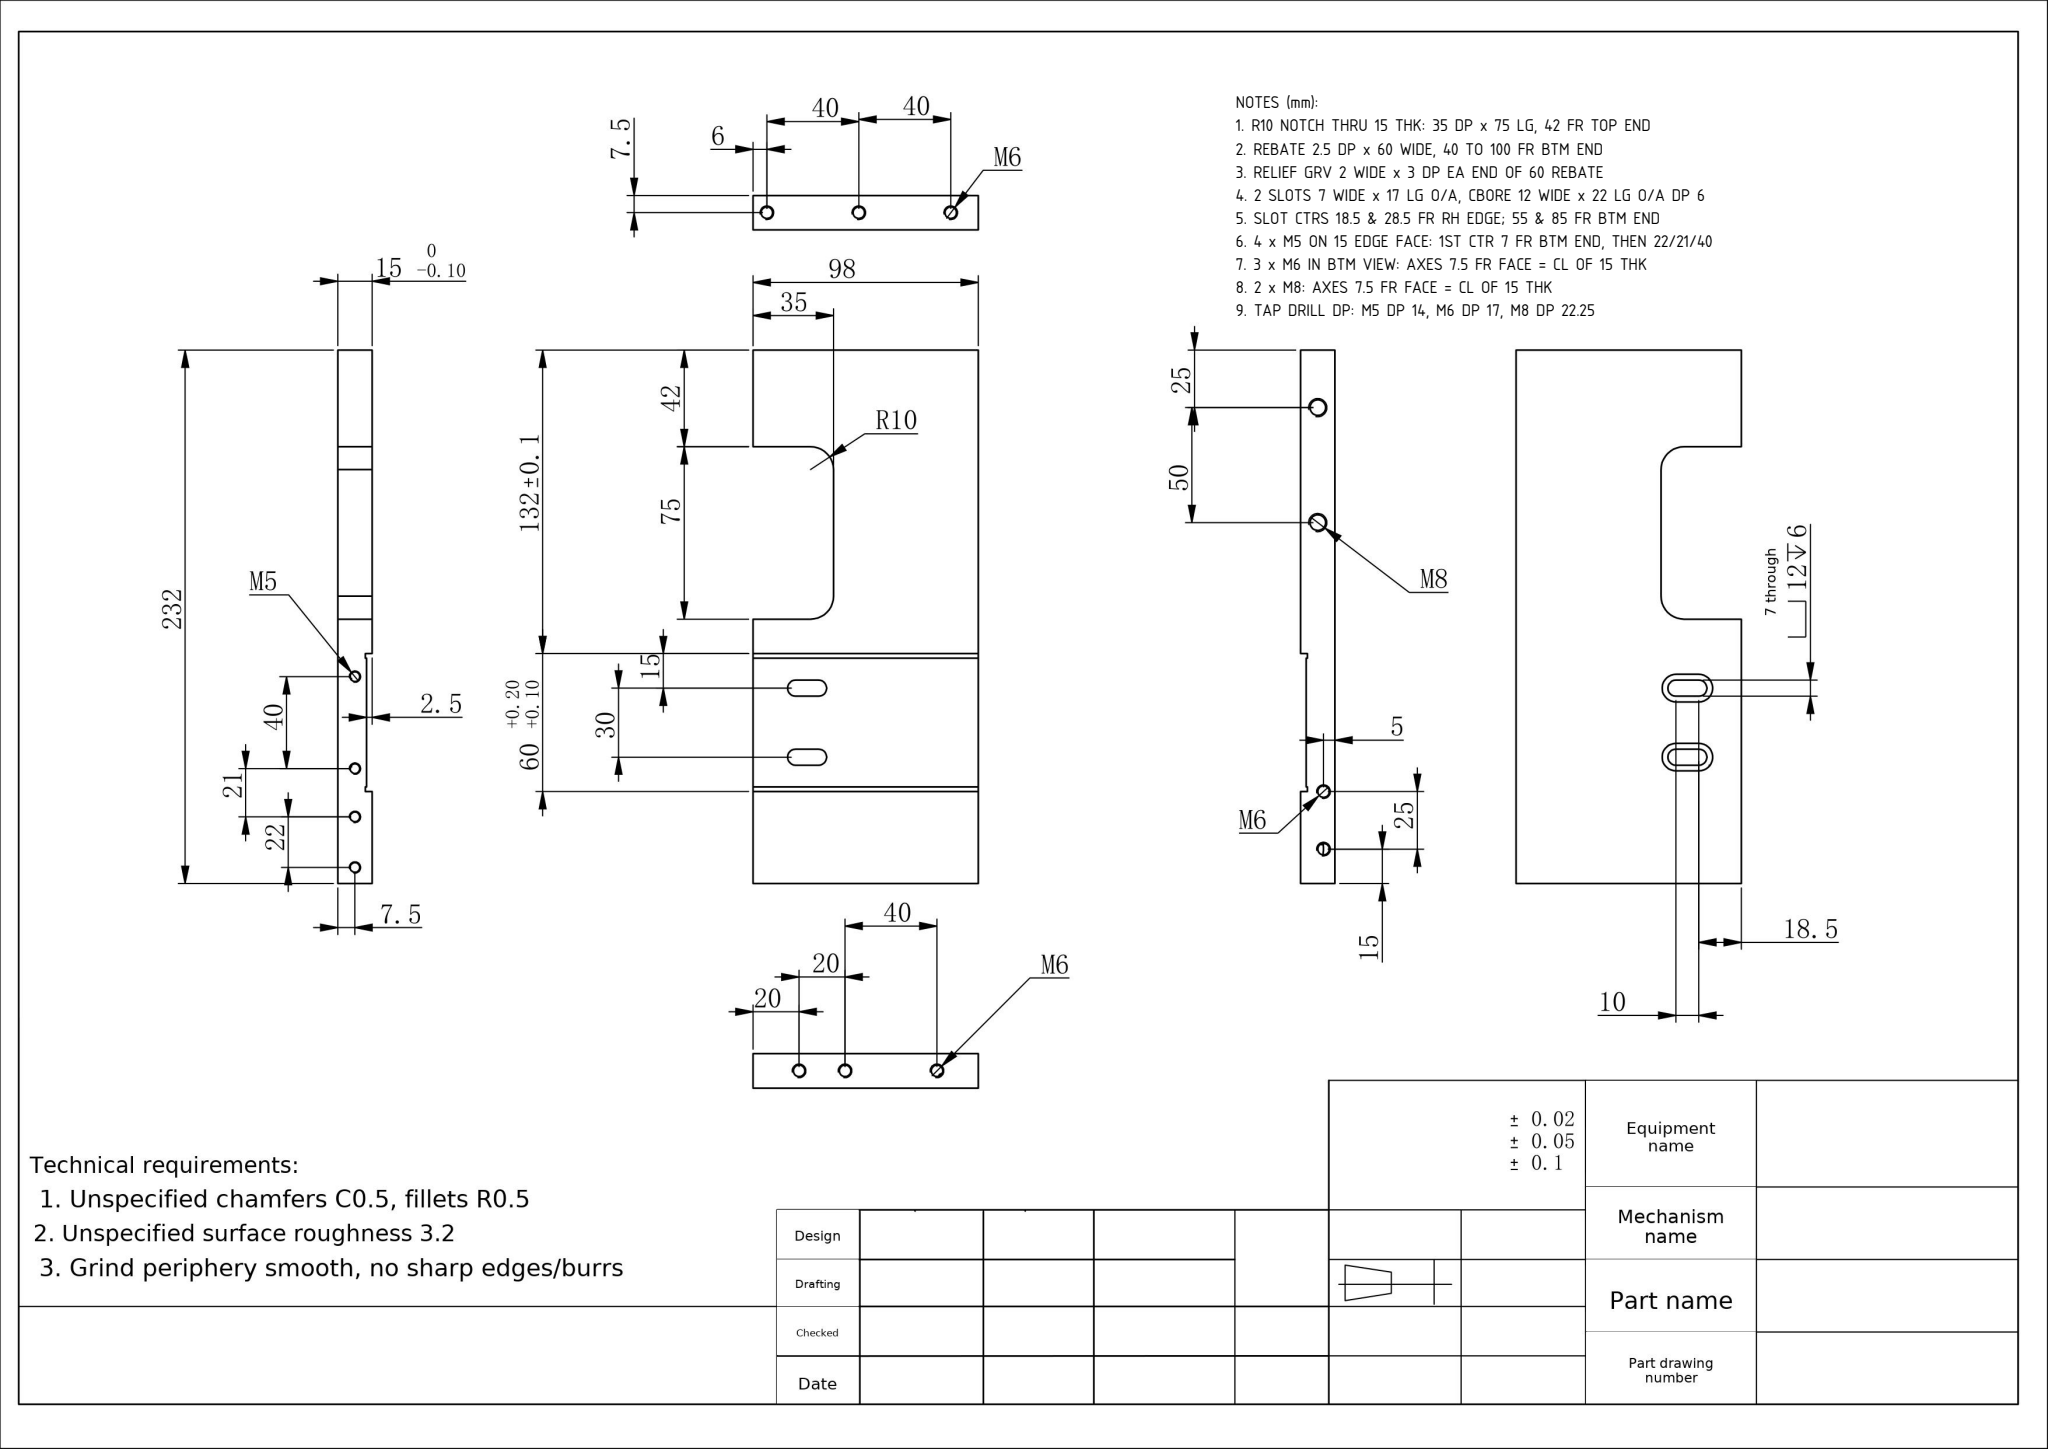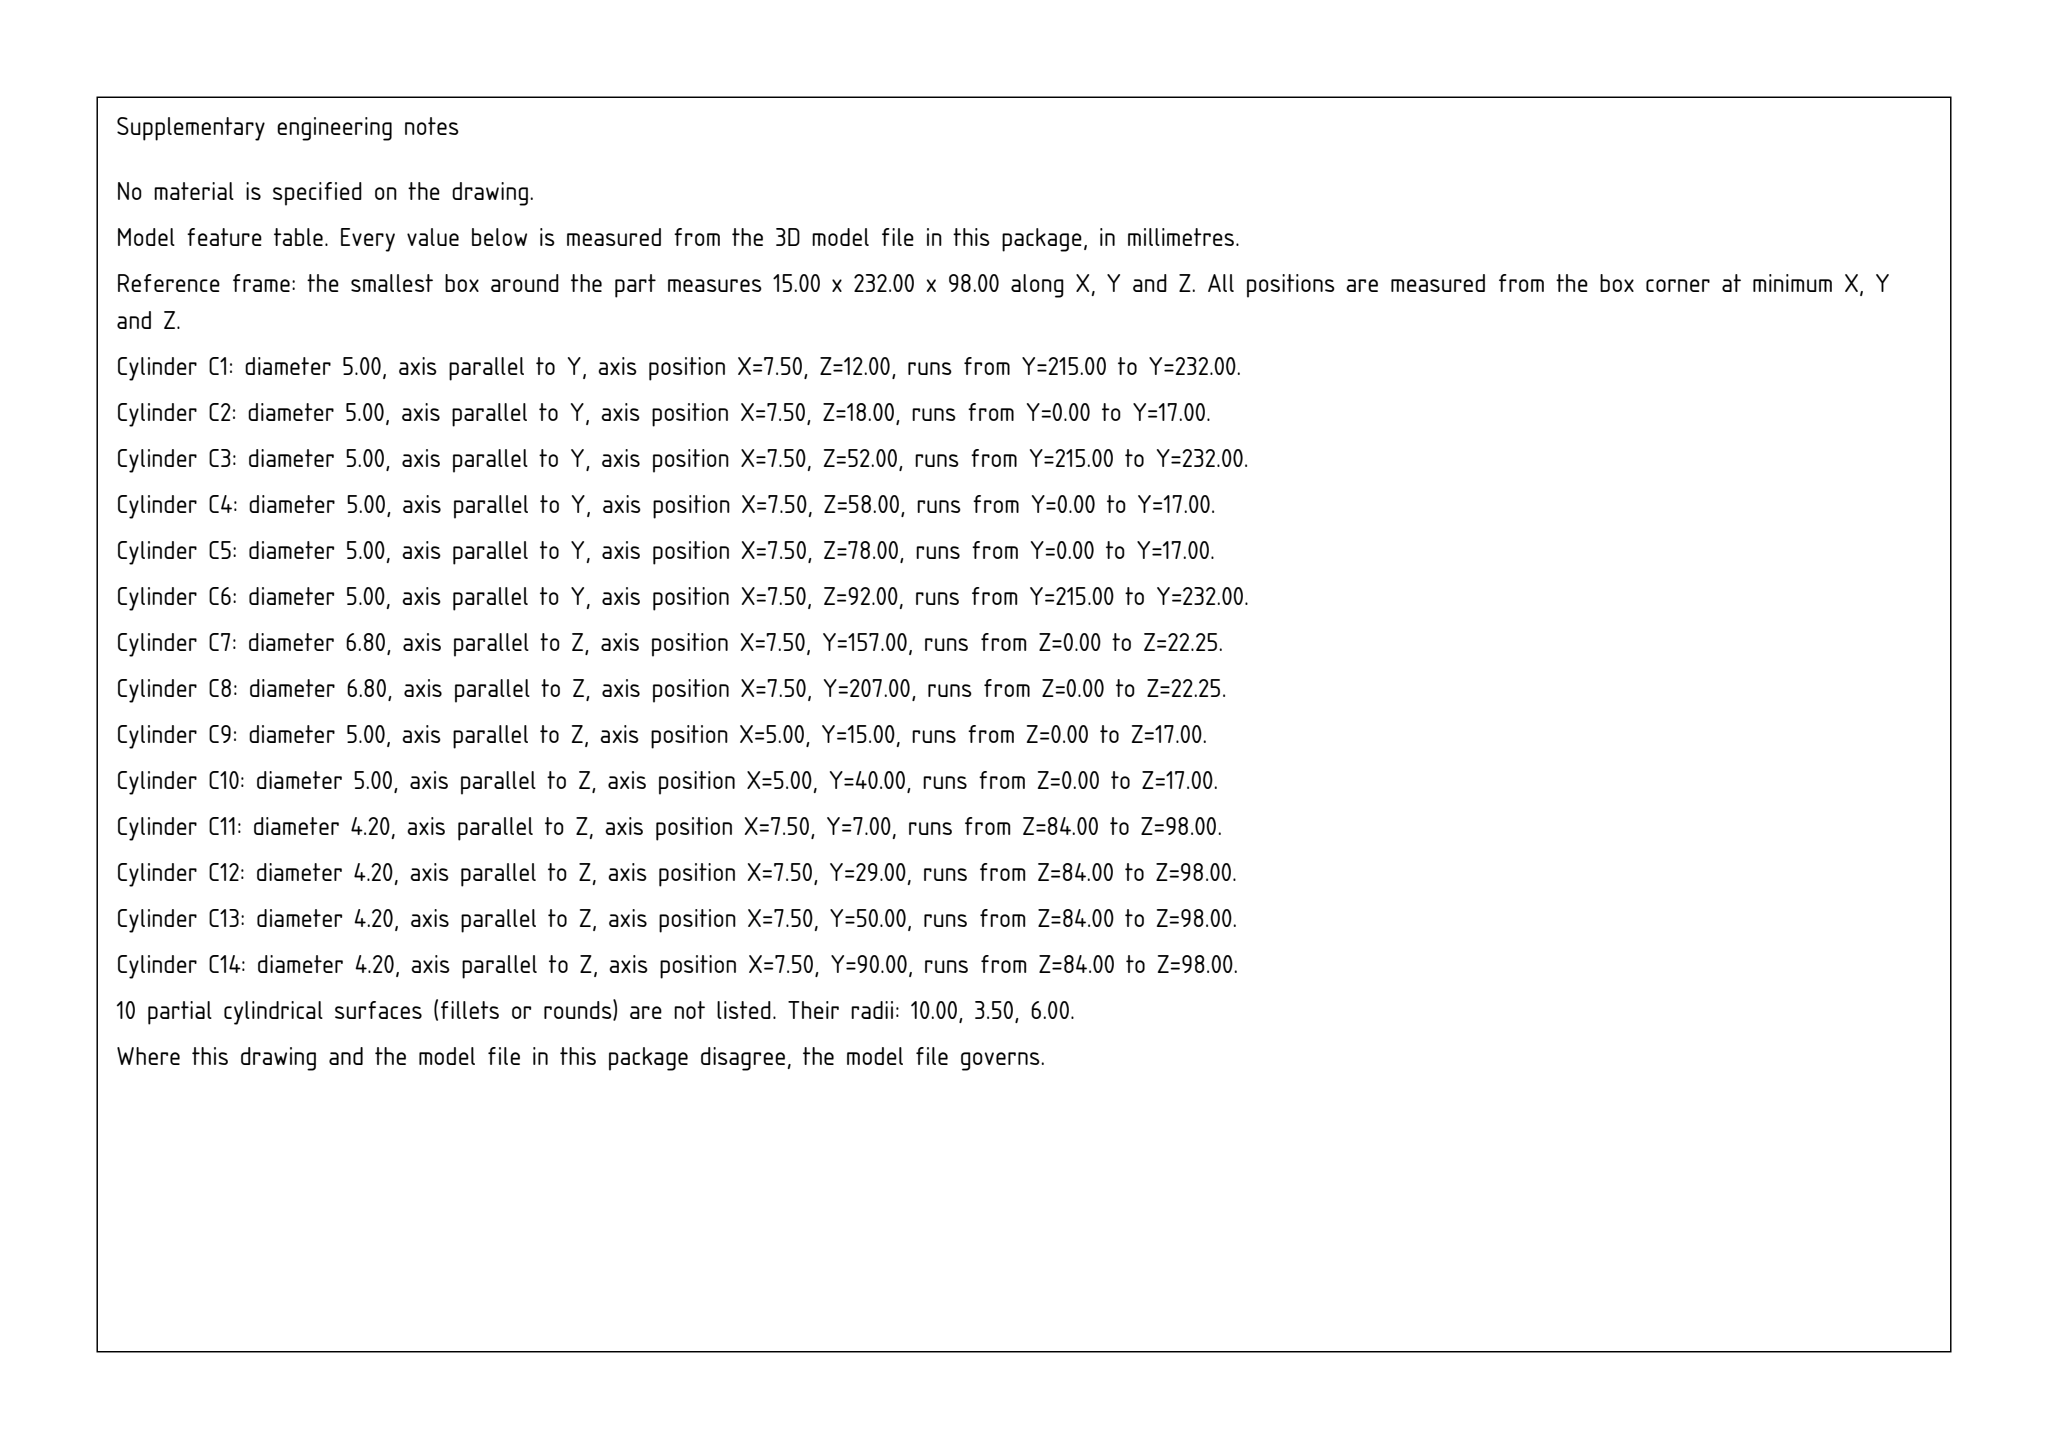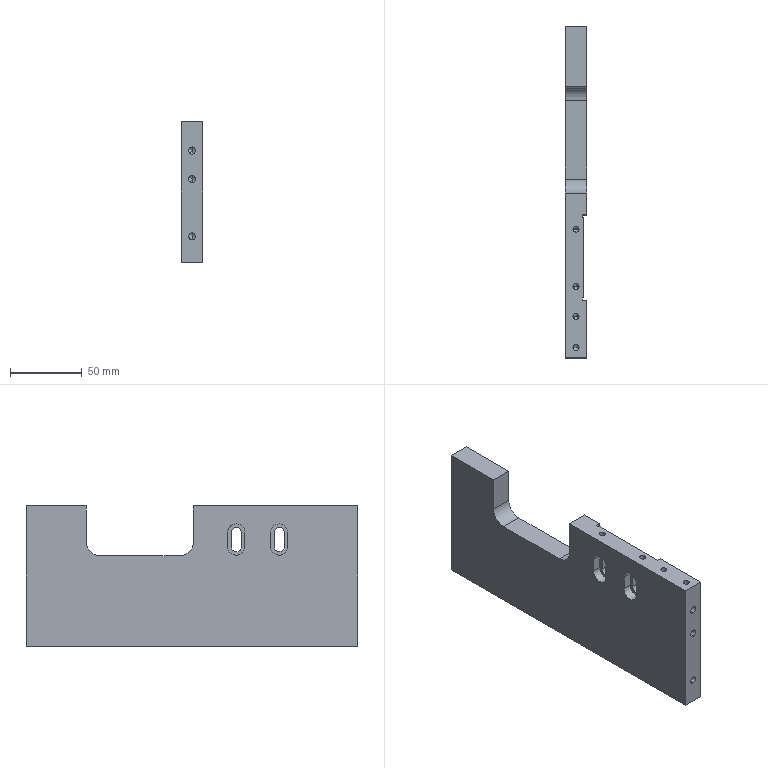Part | SolidWorks | mm | 1 solid | 99 faces | box 15 x 232 x 98 mm | volume 278005 mm3 | cylinder 43 | cone 28 | plane 28 | commonest cylinder face diameters 5 x17 4.2 x8 12 x6 7 x6 6.8 x4 20 x2
Drawing notes:
R10 NOTCH THRU 15 THK: 35 DP x 75 LG, 42 FR TOP END | from the solid: R10 cyls len 15 = full thk; z 63-98 = 35; y 115-190 = 75; 232-190 = 42
REBATE 2.5 DP x 60 WIDE, 40 TO 100 FR BTM END | from the solid: x planes 15 & 12.5 -> 2.5 dp; y planes 40 & 100 -> 60 wide, 40 fr y=0
RELIEF GRV 2 WIDE x 3 DP EA END OF 60 REBATE | from the solid: x plane 12 (2 faces) = 3 dp; y planes 40/42 and 98/100 -> 2 wide
2 SLOTS 7 WIDE x 17 LG O/A, CBORE 12 WIDE x 22 LG O/A DP 6 | from the solid: Ø7 x-axis cyls z=69.5 & 79.5 (10 apart) -> 17 o/a; Ø12 cbore len 6 -> 22 o/a
SLOT CTRS 18.5 & 28.5 FR RH EDGE; 55 & 85 FR BTM END | from the solid: hole axes z=79.5 & 69.5 of 98; y=55 & 85 of 232
4 x M5 ON 15 EDGE FACE: 1ST CTR 7 FR BTM END, THEN 22/21/40 | from the solid: Ø4.2 z-axis holes at y=7,29,50,90, x=7.5 (M5 tap drills)
3 x M6 IN BTM VIEW: AXES 7.5 FR FACE = CL OF 15 THK | from the solid: Ø5.0 y-axis cyls at x=7.5; bbox x=15.0 so 7.5 = mid-thk
2 x M8: AXES 7.5 FR FACE = CL OF 15 THK | from the solid: Ø6.8 z-axis holes at x=7.5, y=157 & 207; bbox x=15
TAP DRILL DP: M5 DP 14, M6 DP 17, M8 DP 22.25 | from the solid: Ø4.2 L=14, Ø5.0 L=17, Ø6.8 L=22.25 cylinders
build123d program:
from build123d import *

# Parameters (mm, degrees)
SKETCH1_W             = 98
SKETCH1_H             = 232
BOSS_EXTRUDE1_DEPTH   = 15
CUT_EXTRUDE1_DEPTH    = 253.295
SKETCH3_W             = 2.5
SKETCH3_H             = 60
CUT_EXTRUDE2_DEPTH    = 120
SKETCH4_W             = 98
SKETCH4_H             = 2
CUT_EXTRUDE3_DEPTH    = 0.5
M6_TAPPED_HOLE1_D     = 5
M6_TAPPED_HOLE1_DEPTH = 17
M6_TAPPED_HOLE1_TIP   = 1.502
M5_TAPPED_HOLE1_D     = 4.2
M5_TAPPED_HOLE1_DEPTH = 14
M5_TAPPED_HOLE1_TIP   = 1.262
M5_TAPPED_HOLE2_D     = 4.2
M5_TAPPED_HOLE2_DEPTH = 14
M5_TAPPED_HOLE2_TIP   = 1.262
M6_TAPPED_HOLE2_D     = 5
M6_TAPPED_HOLE2_DEPTH = 17
M6_TAPPED_HOLE2_TIP   = 1.502
M6_TAPPED_HOLE3_D     = 5
M6_TAPPED_HOLE3_DEPTH = 17
M6_TAPPED_HOLE3_TIP   = 1.502
CUT_EXTRUDE4_DEPTH    = 30
CUT_EXTRUDE5_DEPTH    = 6
M8_TAPPED_HOLE2_D     = 6.8
M8_TAPPED_HOLE2_DEPTH = 22.25
M8_TAPPED_HOLE2_TIP   = 2.043


with BuildPart() as part:
    # Sketch1 → Boss-Extrude1 (new body)
    with BuildSketch(Plane(origin=(0, 0, 0), x_dir=(0, 0, -1), z_dir=(1, 0, 0))):
        with Locations((49, 116)):
            Rectangle(SKETCH1_W, SKETCH1_H)
    extrude(amount=BOSS_EXTRUDE1_DEPTH)

    # Sketch2 → Cut-Extrude1 (cut, through all)
    with BuildSketch(Plane.ZY):
        with BuildLine():
            Line((0, 115), (-25, 115))
            ThreePointArc((-25, 115), (-32.071, 117.929), (-35, 125))
            Line((-35, 125), (-35, 180))
            ThreePointArc((-35, 180), (-32.071, 187.071), (-25, 190))
            Line((-25, 190), (0, 190))
            Line((0, 190), (0, 115))
        make_face()
    extrude(amount=-CUT_EXTRUDE1_DEPTH, mode=Mode.SUBTRACT)

    # Sketch3 → Cut-Extrude2 (cut)
    with BuildSketch(Plane.XY):
        with Locations((13.75, 70)):
            Rectangle(SKETCH3_W, SKETCH3_H)
    extrude(amount=-CUT_EXTRUDE2_DEPTH, mode=Mode.SUBTRACT)

    # Sketch4 → Cut-Extrude3 (cut)
    with BuildSketch(Plane(origin=(12.5, 0, 0), x_dir=(0, 0, -1), z_dir=(1, 0, 0))):
        with Locations((49, 99)):
            Rectangle(SKETCH4_W, SKETCH4_H)
        with Locations((49, 41)):
            Rectangle(SKETCH4_W, SKETCH4_H)
    extrude(amount=-CUT_EXTRUDE3_DEPTH, mode=Mode.SUBTRACT)

    # M6 Tapped Hole1
    with Locations(Plane(origin=(0.3827, 232, 30.22), x_dir=(-1, 0, 0), z_dir=(0, 1, 0))):
        with Locations((-7.117, -116.22), (-7.117, -36.22), (-7.117, -76.22)):
            Hole(M6_TAPPED_HOLE1_D / 2, depth=M6_TAPPED_HOLE1_DEPTH)
            with Locations((0, 0, -(M6_TAPPED_HOLE1_DEPTH + M6_TAPPED_HOLE1_TIP / 2))):  # 118° drill point
                Cone(0, M6_TAPPED_HOLE1_D / 2, M6_TAPPED_HOLE1_TIP, mode=Mode.SUBTRACT)

    # M5 Tapped Hole1
    with Locations(Plane.XY):
        with Locations((7.5, 90), (7.5, 50)):
            Hole(M5_TAPPED_HOLE1_D / 2, depth=M5_TAPPED_HOLE1_DEPTH)
            with Locations((0, 0, -(M5_TAPPED_HOLE1_DEPTH + M5_TAPPED_HOLE1_TIP / 2))):  # 118° drill point
                Cone(0, M5_TAPPED_HOLE1_D / 2, M5_TAPPED_HOLE1_TIP, mode=Mode.SUBTRACT)

    # M5 Tapped Hole2
    with Locations(Plane.XY):
        with Locations((7.5, 29), (7.5, 7)):
            Hole(M5_TAPPED_HOLE2_D / 2, depth=M5_TAPPED_HOLE2_DEPTH)
            with Locations((0, 0, -(M5_TAPPED_HOLE2_DEPTH + M5_TAPPED_HOLE2_TIP / 2))):  # 118° drill point
                Cone(0, M5_TAPPED_HOLE2_D / 2, M5_TAPPED_HOLE2_TIP, mode=Mode.SUBTRACT)

    # M6 Tapped Hole2
    with Locations(Plane(origin=(0, 0, 0), x_dir=(-1, 0, 0), z_dir=(0, -1, 0))):
        with Locations((-7.5, 40), (-7.5, 20), (-7.5, 80)):
            Hole(M6_TAPPED_HOLE2_D / 2, depth=M6_TAPPED_HOLE2_DEPTH)
            with Locations((0, 0, -(M6_TAPPED_HOLE2_DEPTH + M6_TAPPED_HOLE2_TIP / 2))):  # 118° drill point
                Cone(0, M6_TAPPED_HOLE2_D / 2, M6_TAPPED_HOLE2_TIP, mode=Mode.SUBTRACT)

    # M6 Tapped Hole3
    with Locations(Plane(origin=(0, 0, -98), x_dir=(-1, 0, 0), z_dir=(0, 0, -1))):
        with Locations((-5, 15), (-5, 40)):
            Hole(M6_TAPPED_HOLE3_D / 2, depth=M6_TAPPED_HOLE3_DEPTH)
            with Locations((0, 0, -(M6_TAPPED_HOLE3_DEPTH + M6_TAPPED_HOLE3_TIP / 2))):  # 118° drill point
                Cone(0, M6_TAPPED_HOLE3_D / 2, M6_TAPPED_HOLE3_TIP, mode=Mode.SUBTRACT)

    # Sketch16 → Cut-Extrude4 (cut)
    with BuildSketch(Plane.ZY):
        with BuildLine():
            Line((-18.5, 51.5), (-28.5, 51.5))
            ThreePointArc((-28.5, 51.5), (-32, 55), (-28.5, 58.5))
            Line((-28.5, 58.5), (-18.5, 58.5))
            ThreePointArc((-18.5, 58.5), (-15, 55), (-18.5, 51.5))
        make_face()
        with BuildLine():
            Line((-18.5, 81.5), (-28.5, 81.5))
            ThreePointArc((-28.5, 81.5), (-32, 85), (-28.5, 88.5))
            Line((-28.5, 88.5), (-18.5, 88.5))
            ThreePointArc((-18.5, 88.5), (-15, 85), (-18.5, 81.5))
        make_face()
    extrude(amount=-CUT_EXTRUDE4_DEPTH, mode=Mode.SUBTRACT)

    # Sketch17 → Cut-Extrude5 (cut)
    with BuildSketch(Plane.ZY):
        with BuildLine():
            Line((-28.5, 79), (-18.5, 79))
            ThreePointArc((-18.5, 79), (-12.5, 85), (-18.5, 91))
            Line((-18.5, 91), (-28.5, 91))
            ThreePointArc((-28.5, 91), (-34.5, 85), (-28.5, 79))
        make_face()
        with BuildLine():
            Line((-28.5, 49), (-18.5, 49))
            ThreePointArc((-18.5, 49), (-12.5, 55), (-18.5, 61))
            Line((-18.5, 61), (-28.5, 61))
            ThreePointArc((-28.5, 61), (-34.5, 55), (-28.5, 49))
        make_face()
    extrude(amount=-CUT_EXTRUDE5_DEPTH, mode=Mode.SUBTRACT)

    # M8 Tapped Hole2
    with Locations(Plane(origin=(0, 0, -98), x_dir=(-1, 0, 0), z_dir=(0, 0, -1))):
        with Locations((-7.5, 157), (-7.5, 207)):
            Hole(M8_TAPPED_HOLE2_D / 2, depth=M8_TAPPED_HOLE2_DEPTH)
            with Locations((0, 0, -(M8_TAPPED_HOLE2_DEPTH + M8_TAPPED_HOLE2_TIP / 2))):  # 118° drill point
                Cone(0, M8_TAPPED_HOLE2_D / 2, M8_TAPPED_HOLE2_TIP, mode=Mode.SUBTRACT)


solid = part.part